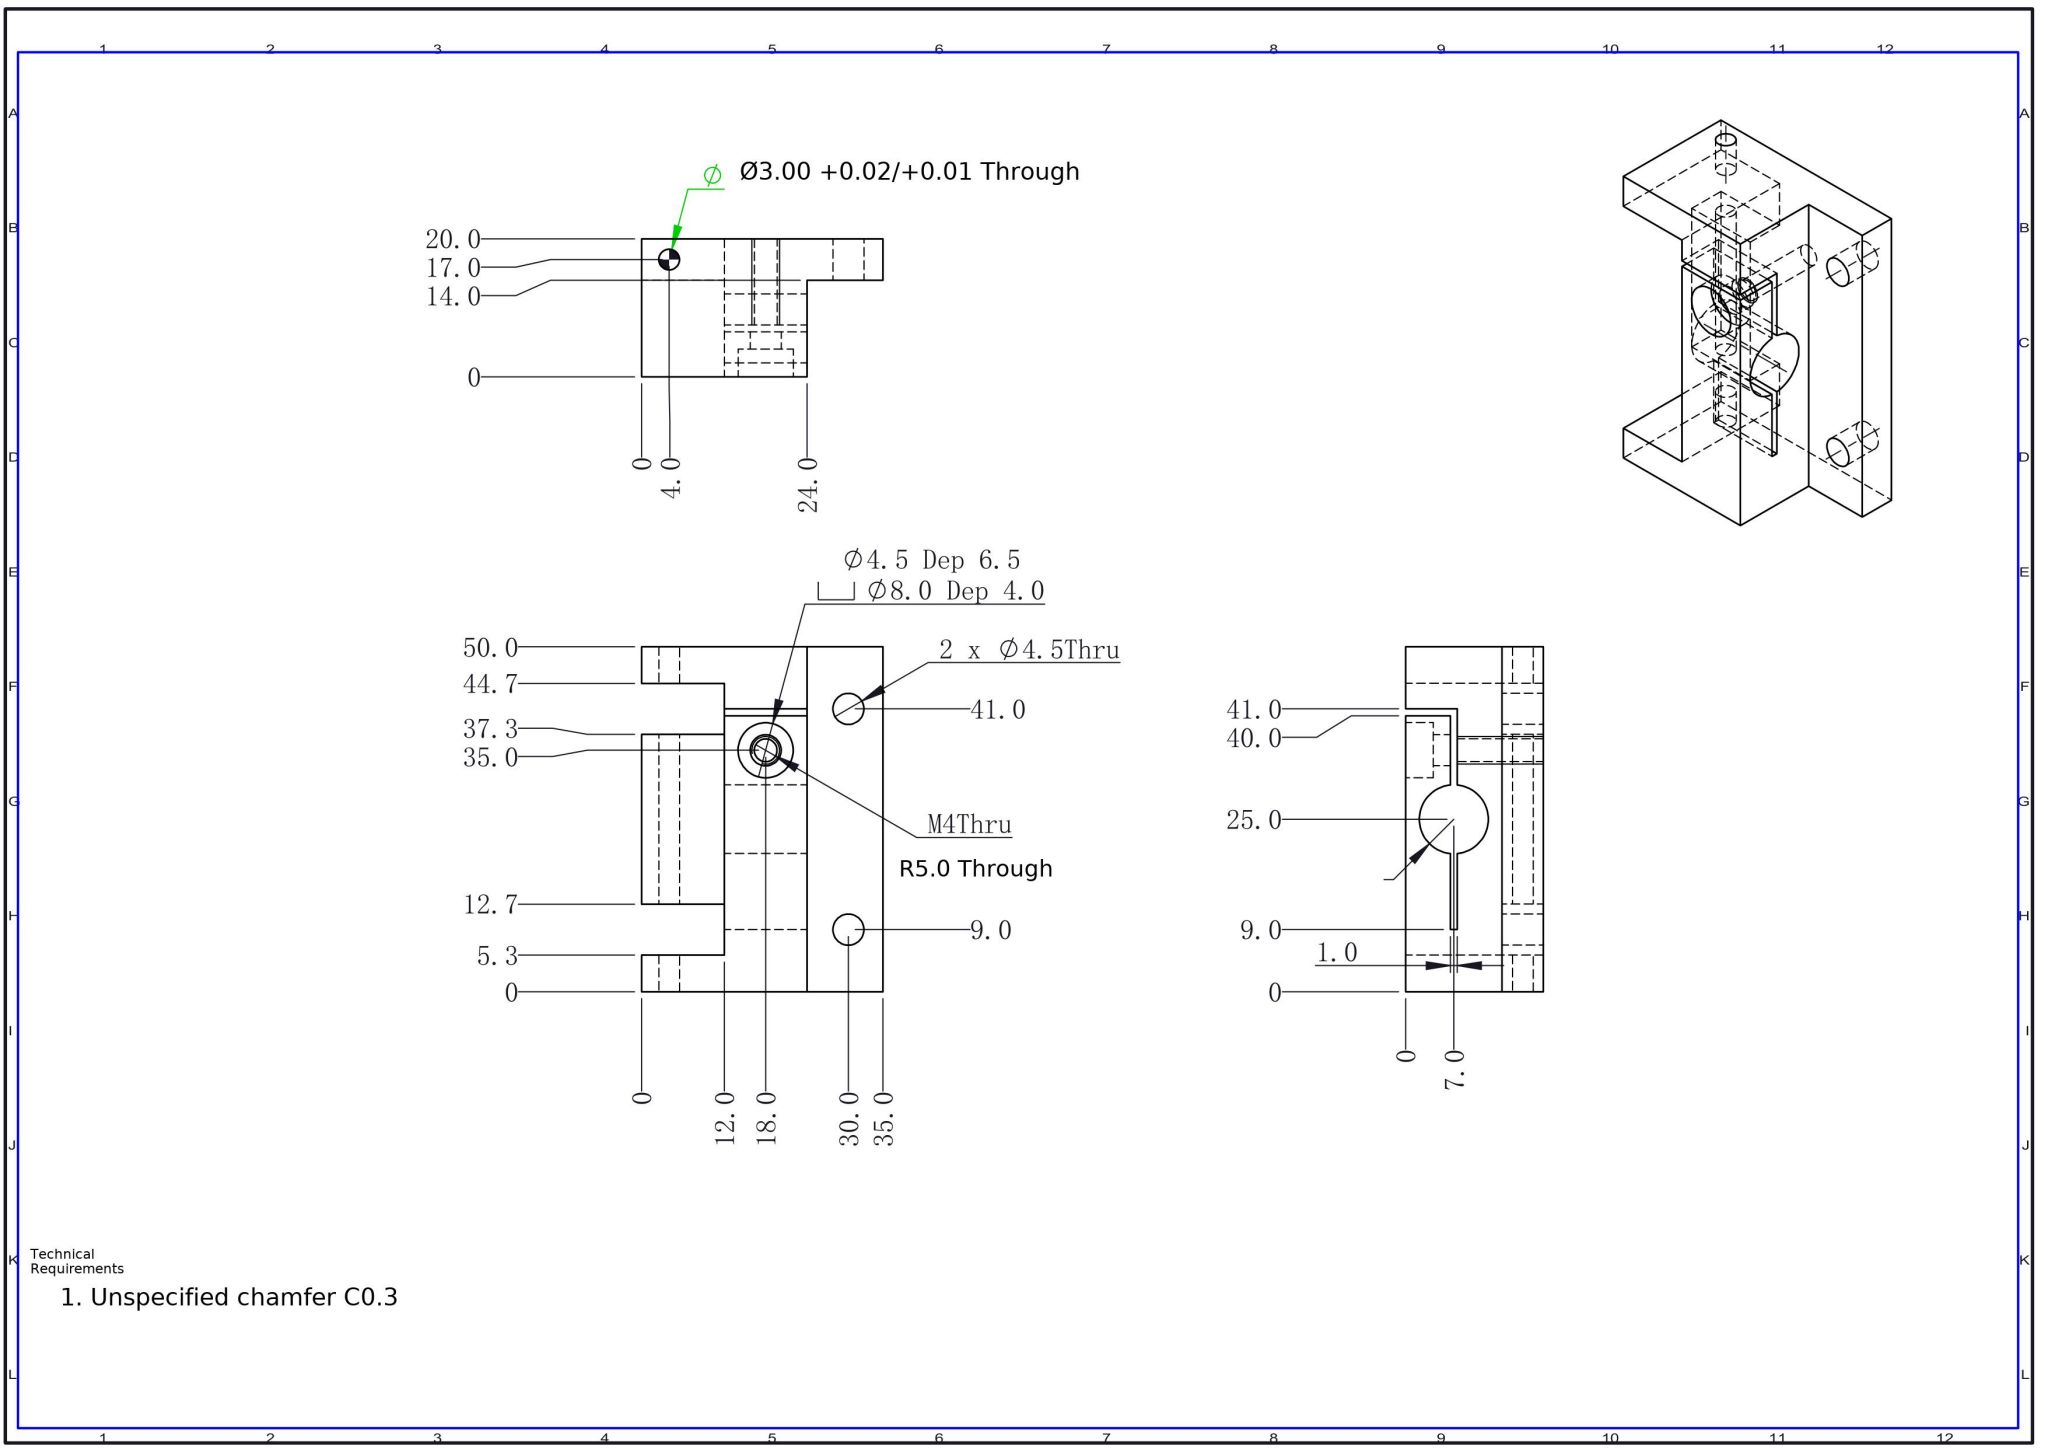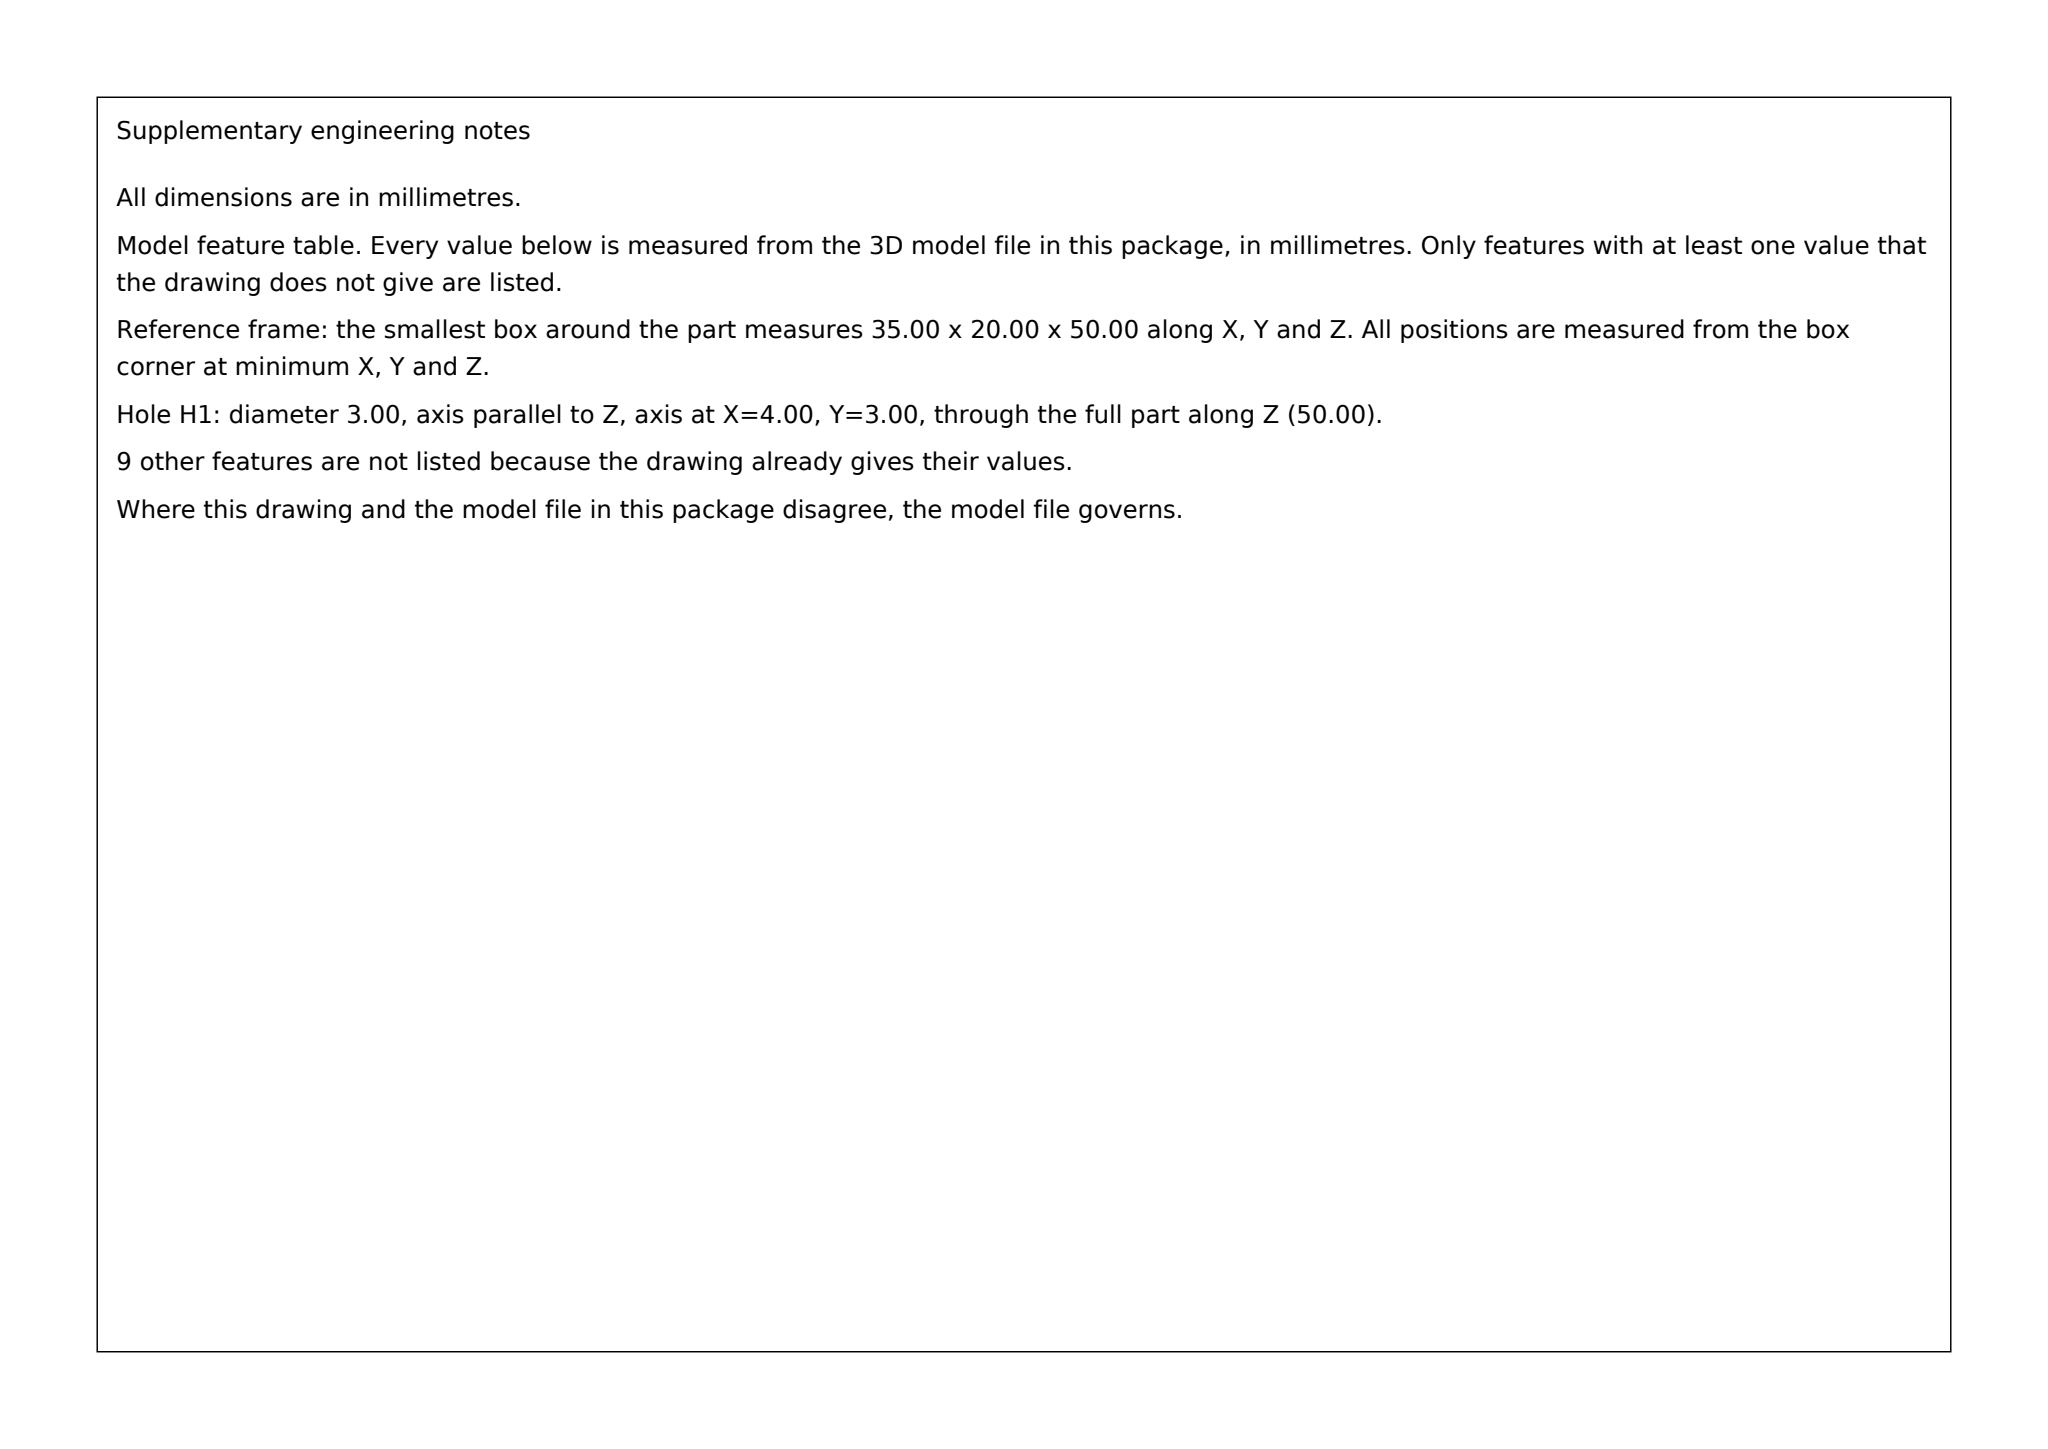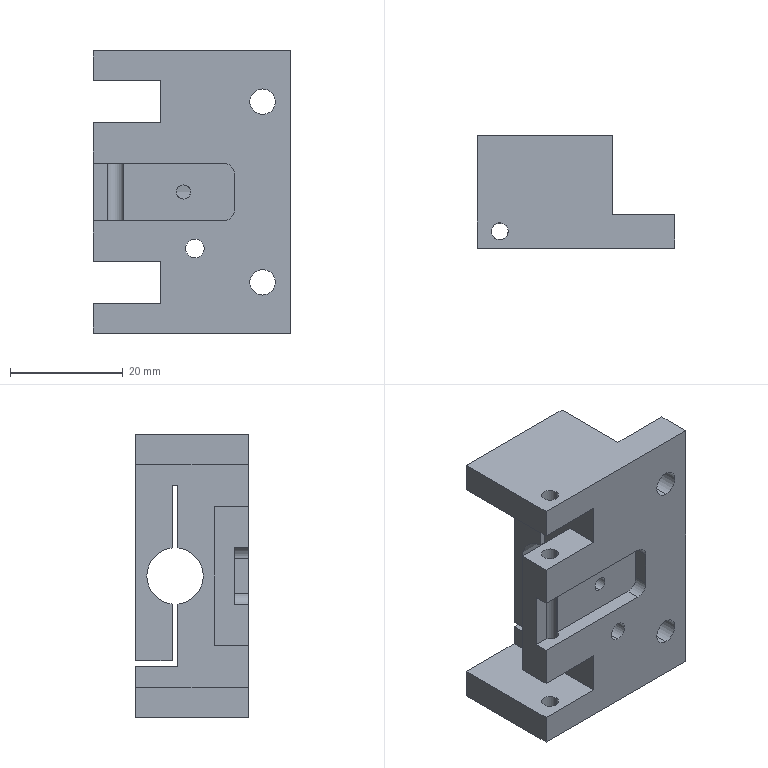Part | SolidWorks | mm | 1 solid | 52 faces | box 35 x 20 x 50 mm | volume 16904 mm3 | plane 30 | cylinder 22 | commonest cylinder face diameters 4.5 x6 3 x6 2.5 x2 3.3 x2 8 x2 10 x2 4 x2